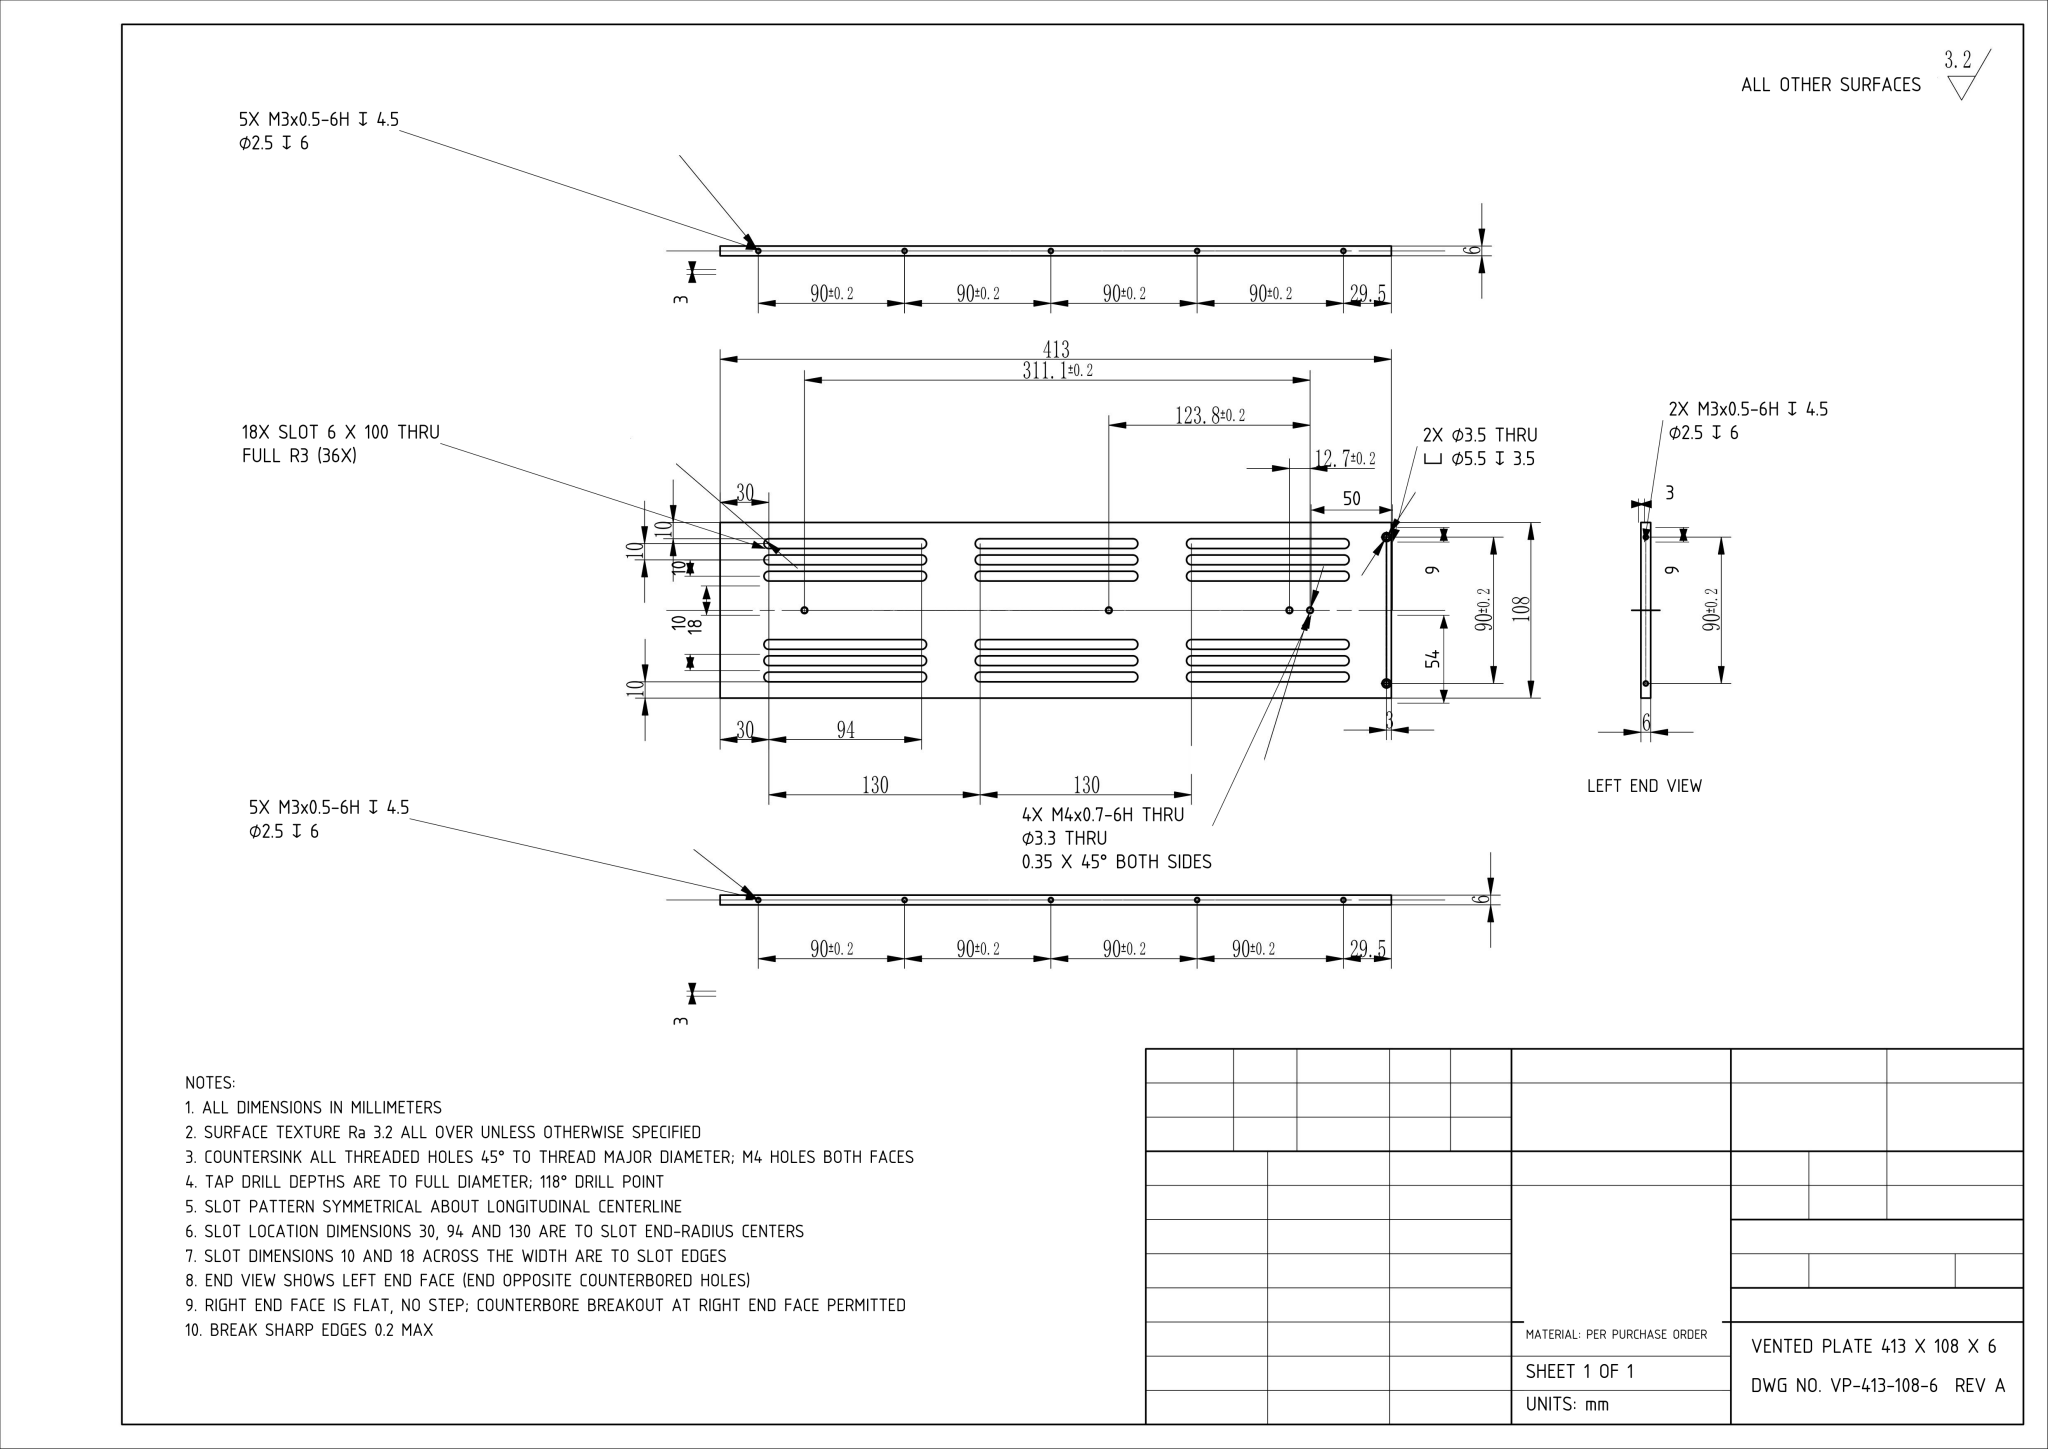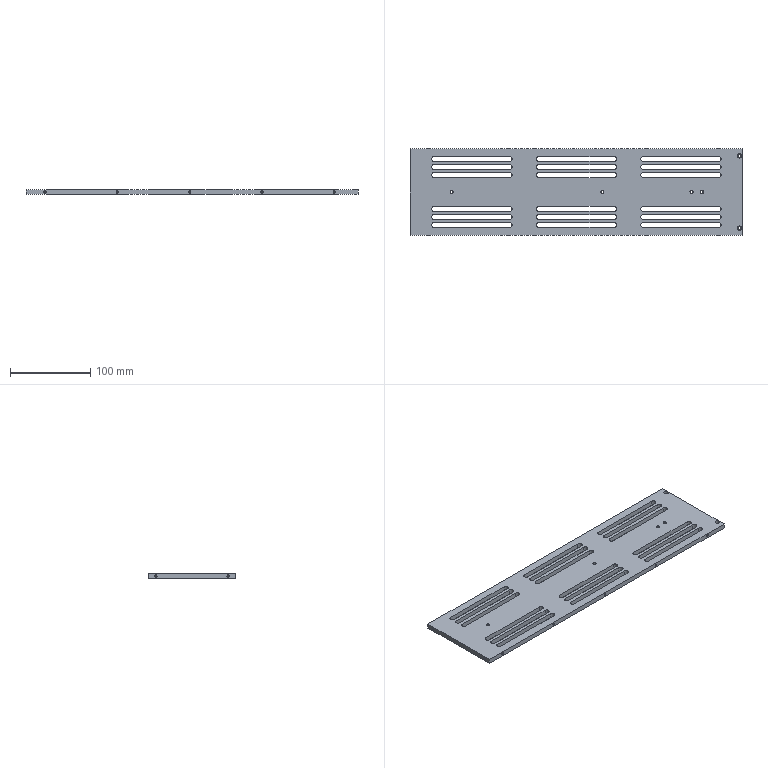Part | NX | mm | 1 solid | 132 faces | box 413 x 108 x 6 mm | volume 202862 mm3 | cylinder 56 | plane 44 | cone 32 | commonest cylinder face diameters 6 x36 2.5 x12 3.3 x4 3.5 x2 5.5 x2